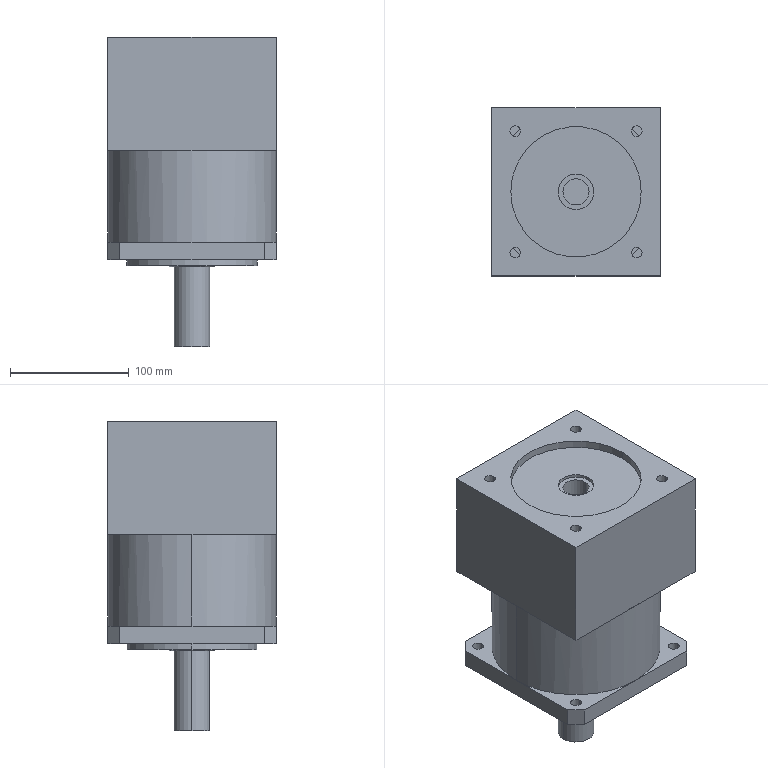Component | SolidWorks | Reducer(CHINT)ZDH-120-L1-R10-1 | 1 solid | 62 faces | volume 3439363 mm3 | plane 32 | cylinder 28 | cone 2 | commonest cylinder face diameters 9 x16 30 x4 22.02 x2 110.02 x2 142 x2 110 x2